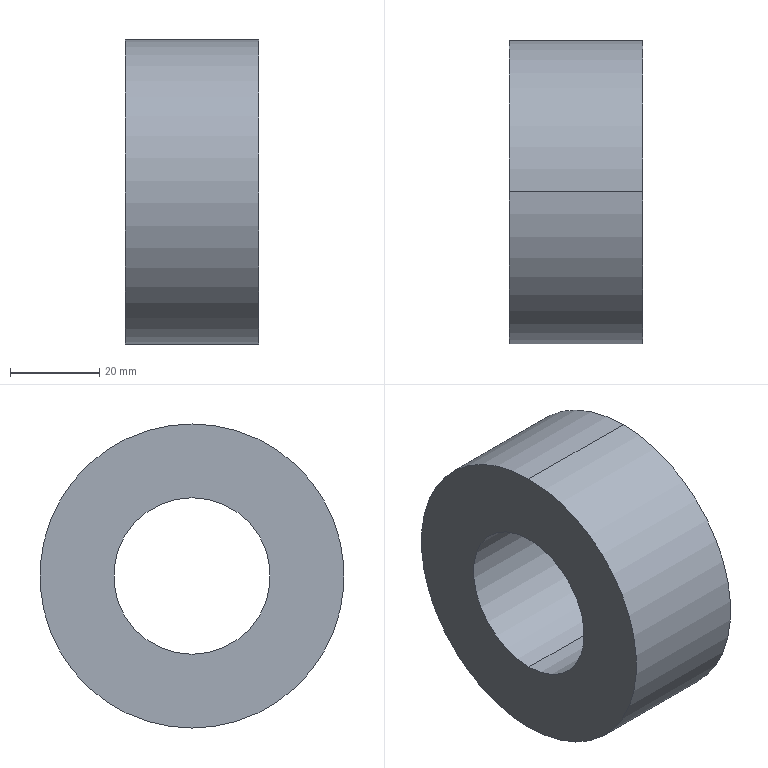Component | SolidWorks | SmallThrustBearing-1 | 1 solid | 8 faces | box 29.79 x 68 x 68 mm | volume 79399 mm3 | cylinder 4 | cone 2 | plane 2 | commonest cylinder face diameters 35 x2 68 x2
build123d program:
from build123d import *

# Parameters (mm, degrees)
SKETCH1_R           = 34
SKETCH1_R_2         = 17.5
BOSS_EXTRUDE1_DEPTH = 29.79
CHAMFER1_SIZE       = 1.5


with BuildPart() as part:
    # Sketch1 → Boss-Extrude1 (new body)
    with BuildSketch(Plane(origin=(0, 0, 0), x_dir=(0, 0, -1), z_dir=(1, 0, 0))):
        Circle(SKETCH1_R)
        Circle(SKETCH1_R_2, mode=Mode.SUBTRACT)
    extrude(amount=BOSS_EXTRUDE1_DEPTH)

    # Chamfer1
    chamfer1_edges = [part.edges().sort_by_distance(p)[0] for p in [
        (29.79, 0, 17.5),
    ]]
    chamfer(chamfer1_edges, length=CHAMFER1_SIZE)


solid = part.part

# Placed as in the assembly
solid = solid.moved(Location((459.733, 15.31, -240), (0, 0, 0)))
STEP:
#1=COLOUR_RGB('',0.7922,0.8196,0.9333);
#2=FILL_AREA_STYLE_COLOUR('',#1);
#3=FILL_AREA_STYLE('',(#2));
#4=SURFACE_STYLE_FILL_AREA(#3);
#5=SURFACE_SIDE_STYLE('',(#4));
#6=SURFACE_STYLE_USAGE(.BOTH.,#5);
#7=PRESENTATION_STYLE_ASSIGNMENT((#6));
#8=CARTESIAN_POINT('',(19.213,0.6028,-8.76));
#9=VERTEX_POINT('',#8);
#10=CARTESIAN_POINT('',(19.213,0.6028,-10.138));
#11=VERTEX_POINT('',#10);
#12=CARTESIAN_POINT('',(19.213,0.6028,-9.449));
#13=DIRECTION('',(1.,0.,0.));
#14=DIRECTION('',(0.,0.,-1.));
#15=AXIS2_PLACEMENT_3D('',#12,#13,#14);
#16=CIRCLE('',#15,0.689);
#17=EDGE_CURVE('',#9,#11,#16,.T.);
#18=ORIENTED_EDGE('',*,*,#17,.F.);
#19=CARTESIAN_POINT('',(19.273,0.6028,-8.701));
#20=VERTEX_POINT('',#19);
#21=CARTESIAN_POINT('',(19.213,0.6028,-8.76));
#22=DIRECTION('',(0.7071,0.,0.7071));
#23=VECTOR('',#22,39.37);
#24=LINE('',#21,#23);
#25=EDGE_CURVE('',#9,#20,#24,.T.);
#26=ORIENTED_EDGE('',*,*,#25,.T.);
#27=CARTESIAN_POINT('',(19.273,0.6028,-10.197));
#28=VERTEX_POINT('',#27);
#29=CARTESIAN_POINT('',(19.273,0.6028,-9.449));
#30=DIRECTION('',(-1.,0.,0.));
#31=DIRECTION('',(0.,0.,-1.));
#32=AXIS2_PLACEMENT_3D('',#29,#30,#31);
#33=CIRCLE('',#32,0.748);
#34=EDGE_CURVE('',#28,#20,#33,.T.);
#35=ORIENTED_EDGE('',*,*,#34,.F.);
#36=CARTESIAN_POINT('',(19.213,0.6028,-10.138));
#37=DIRECTION('',(0.7071,0.,-0.7071));
#38=VECTOR('',#37,39.37);
#39=LINE('',#36,#38);
#40=EDGE_CURVE('',#11,#28,#39,.T.);
#41=ORIENTED_EDGE('',*,*,#40,.F.);
#42=EDGE_LOOP('',(#18,#26,#35,#41));
#43=FACE_OUTER_BOUND('',#42,.T.);
#44=CARTESIAN_POINT('',(19.213,0.6028,-9.449));
#45=DIRECTION('',(1.,0.,0.));
#46=DIRECTION('',(0.,0.,-1.));
#47=AXIS2_PLACEMENT_3D('',#44,#45,#46);
#48=CONICAL_SURFACE('',#47,0.689,0.7854);
#49=ADVANCED_FACE('',(#43),#48,.F.);
#50=ORIENTED_EDGE('',*,*,#17,.T.);
#51=CARTESIAN_POINT('',(18.1,0.6028,-10.138));
#52=VERTEX_POINT('',#51);
#53=CARTESIAN_POINT('',(19.273,0.6028,-10.138));
#54=DIRECTION('',(-1.,0.,0.));
#55=VECTOR('',#54,39.37);
#56=LINE('',#53,#55);
#57=EDGE_CURVE('',#11,#52,#56,.T.);
#58=ORIENTED_EDGE('',*,*,#57,.T.);
#59=CARTESIAN_POINT('',(18.1,0.6028,-8.76));
#60=VERTEX_POINT('',#59);
#61=CARTESIAN_POINT('',(18.1,0.6028,-9.449));
#62=DIRECTION('',(1.,0.,0.));
#63=DIRECTION('',(0.,0.,-1.));
#64=AXIS2_PLACEMENT_3D('',#61,#62,#63);
#65=CIRCLE('',#64,0.689);
#66=EDGE_CURVE('',#60,#52,#65,.T.);
#67=ORIENTED_EDGE('',*,*,#66,.F.);
#68=CARTESIAN_POINT('',(19.273,0.6028,-8.76));
#69=DIRECTION('',(-1.,0.,0.));
#70=VECTOR('',#69,39.37);
#71=LINE('',#68,#70);
#72=EDGE_CURVE('',#9,#60,#71,.T.);
#73=ORIENTED_EDGE('',*,*,#72,.F.);
#74=EDGE_LOOP('',(#50,#58,#67,#73));
#75=FACE_OUTER_BOUND('',#74,.T.);
#76=CARTESIAN_POINT('',(19.273,0.6028,-9.449));
#77=DIRECTION('',(-1.,0.,0.));
#78=DIRECTION('',(0.,0.,1.));
#79=AXIS2_PLACEMENT_3D('',#76,#77,#78);
#80=CYLINDRICAL_SURFACE('',#79,0.689);
#81=ADVANCED_FACE('',(#75),#80,.F.);
#82=CARTESIAN_POINT('',(19.273,0.6028,-10.787));
#83=VERTEX_POINT('',#82);
#84=CARTESIAN_POINT('',(19.273,0.6028,-8.11));
#85=VERTEX_POINT('',#84);
#86=CARTESIAN_POINT('',(19.273,0.6028,-9.449));
#87=DIRECTION('',(1.,0.,0.));
#88=DIRECTION('',(0.,0.,-1.));
#89=AXIS2_PLACEMENT_3D('',#86,#87,#88);
#90=CIRCLE('',#89,1.339);
#91=EDGE_CURVE('',#83,#85,#90,.T.);
#92=ORIENTED_EDGE('',*,*,#91,.F.);
#93=CARTESIAN_POINT('',(18.1,0.6028,-10.787));
#94=VERTEX_POINT('',#93);
#95=CARTESIAN_POINT('',(19.273,0.6028,-10.787));
#96=DIRECTION('',(-1.,0.,0.));
#97=VECTOR('',#96,39.37);
#98=LINE('',#95,#97);
#99=EDGE_CURVE('',#83,#94,#98,.T.);
#100=ORIENTED_EDGE('',*,*,#99,.T.);
#101=CARTESIAN_POINT('',(18.1,0.6028,-8.11));
#102=VERTEX_POINT('',#101);
#103=CARTESIAN_POINT('',(18.1,0.6028,-9.449));
#104=DIRECTION('',(1.,0.,0.));
#105=DIRECTION('',(0.,0.,-1.));
#106=AXIS2_PLACEMENT_3D('',#103,#104,#105);
#107=CIRCLE('',#106,1.339);
#108=EDGE_CURVE('',#94,#102,#107,.T.);
#109=ORIENTED_EDGE('',*,*,#108,.T.);
#110=CARTESIAN_POINT('',(19.273,0.6028,-8.11));
#111=DIRECTION('',(-1.,0.,0.));
#112=VECTOR('',#111,39.37);
#113=LINE('',#110,#112);
#114=EDGE_CURVE('',#85,#102,#113,.T.);
#115=ORIENTED_EDGE('',*,*,#114,.F.);
#116=EDGE_LOOP('',(#92,#100,#109,#115));
#117=FACE_OUTER_BOUND('',#116,.T.);
#118=CARTESIAN_POINT('',(19.273,0.6028,-9.449));
#119=DIRECTION('',(-1.,0.,0.));
#120=DIRECTION('',(0.,0.,1.));
#121=AXIS2_PLACEMENT_3D('',#118,#119,#120);
#122=CYLINDRICAL_SURFACE('',#121,1.339);
#123=ADVANCED_FACE('',(#117),#122,.T.);
#124=ORIENTED_EDGE('',*,*,#34,.T.);
#125=CARTESIAN_POINT('',(19.273,0.6028,-9.449));
#126=DIRECTION('',(-1.,0.,0.));
#127=DIRECTION('',(0.,0.,-1.));
#128=AXIS2_PLACEMENT_3D('',#125,#126,#127);
#129=CIRCLE('',#128,0.748);
#130=EDGE_CURVE('',#20,#28,#129,.T.);
#131=ORIENTED_EDGE('',*,*,#130,.T.);
#132=EDGE_LOOP('',(#124,#131));
#133=FACE_BOUND('',#132,.T.);
#134=CARTESIAN_POINT('',(19.273,0.6028,-9.449));
#135=DIRECTION('',(1.,0.,0.));
#136=DIRECTION('',(0.,0.,-1.));
#137=AXIS2_PLACEMENT_3D('',#134,#135,#136);
#138=CIRCLE('',#137,1.339);
#139=EDGE_CURVE('',#85,#83,#138,.T.);
#140=ORIENTED_EDGE('',*,*,#139,.T.);
#141=ORIENTED_EDGE('',*,*,#91,.T.);
#142=EDGE_LOOP('',(#140,#141));
#143=FACE_OUTER_BOUND('',#142,.T.);
#144=CARTESIAN_POINT('',(19.273,0.6028,-9.449));
#145=DIRECTION('',(1.,0.,0.));
#146=DIRECTION('',(0.,0.,-1.));
#147=AXIS2_PLACEMENT_3D('',#144,#145,#146);
#148=PLANE('',#147);
#149=ADVANCED_FACE('',(#133,#143),#148,.T.);
#150=CARTESIAN_POINT('',(18.1,0.6028,-9.449));
#151=DIRECTION('',(1.,0.,0.));
#152=DIRECTION('',(0.,0.,-1.));
#153=AXIS2_PLACEMENT_3D('',#150,#151,#152);
#154=CIRCLE('',#153,1.339);
#155=EDGE_CURVE('',#102,#94,#154,.T.);
#156=ORIENTED_EDGE('',*,*,#155,.F.);
#157=ORIENTED_EDGE('',*,*,#108,.F.);
#158=EDGE_LOOP('',(#156,#157));
#159=FACE_OUTER_BOUND('',#158,.T.);
#160=ORIENTED_EDGE('',*,*,#66,.T.);
#161=CARTESIAN_POINT('',(18.1,0.6028,-9.449));
#162=DIRECTION('',(1.,0.,0.));
#163=DIRECTION('',(0.,0.,-1.));
#164=AXIS2_PLACEMENT_3D('',#161,#162,#163);
#165=CIRCLE('',#164,0.689);
#166=EDGE_CURVE('',#52,#60,#165,.T.);
#167=ORIENTED_EDGE('',*,*,#166,.T.);
#168=EDGE_LOOP('',(#160,#167));
#169=FACE_BOUND('',#168,.T.);
#170=CARTESIAN_POINT('',(18.1,0.6028,-9.449));
#171=DIRECTION('',(1.,0.,0.));
#172=DIRECTION('',(0.,0.,-1.));
#173=AXIS2_PLACEMENT_3D('',#170,#171,#172);
#174=PLANE('',#173);
#175=ADVANCED_FACE('',(#159,#169),#174,.F.);
#176=ORIENTED_EDGE('',*,*,#99,.F.);
#177=ORIENTED_EDGE('',*,*,#139,.F.);
#178=ORIENTED_EDGE('',*,*,#114,.T.);
#179=ORIENTED_EDGE('',*,*,#155,.T.);
#180=EDGE_LOOP('',(#176,#177,#178,#179));
#181=FACE_OUTER_BOUND('',#180,.T.);
#182=CARTESIAN_POINT('',(19.273,0.6028,-9.449));
#183=DIRECTION('',(-1.,0.,0.));
#184=DIRECTION('',(0.,0.,1.));
#185=AXIS2_PLACEMENT_3D('',#182,#183,#184);
#186=CYLINDRICAL_SURFACE('',#185,1.339);
#187=ADVANCED_FACE('',(#181),#186,.T.);
#188=ORIENTED_EDGE('',*,*,#57,.F.);
#189=CARTESIAN_POINT('',(19.213,0.6028,-9.449));
#190=DIRECTION('',(1.,0.,0.));
#191=DIRECTION('',(0.,0.,-1.));
#192=AXIS2_PLACEMENT_3D('',#189,#190,#191);
#193=CIRCLE('',#192,0.689);
#194=EDGE_CURVE('',#11,#9,#193,.T.);
#195=ORIENTED_EDGE('',*,*,#194,.T.);
#196=ORIENTED_EDGE('',*,*,#72,.T.);
#197=ORIENTED_EDGE('',*,*,#166,.F.);
#198=EDGE_LOOP('',(#188,#195,#196,#197));
#199=FACE_OUTER_BOUND('',#198,.T.);
#200=CARTESIAN_POINT('',(19.273,0.6028,-9.449));
#201=DIRECTION('',(-1.,0.,0.));
#202=DIRECTION('',(0.,0.,1.));
#203=AXIS2_PLACEMENT_3D('',#200,#201,#202);
#204=CYLINDRICAL_SURFACE('',#203,0.689);
#205=ADVANCED_FACE('',(#199),#204,.F.);
#206=ORIENTED_EDGE('',*,*,#25,.F.);
#207=ORIENTED_EDGE('',*,*,#194,.F.);
#208=ORIENTED_EDGE('',*,*,#40,.T.);
#209=ORIENTED_EDGE('',*,*,#130,.F.);
#210=EDGE_LOOP('',(#206,#207,#208,#209));
#211=FACE_OUTER_BOUND('',#210,.T.);
#212=CARTESIAN_POINT('',(19.213,0.6028,-9.449));
#213=DIRECTION('',(1.,0.,0.));
#214=DIRECTION('',(0.,0.,-1.));
#215=AXIS2_PLACEMENT_3D('',#212,#213,#214);
#216=CONICAL_SURFACE('',#215,0.689,0.7854);
#217=ADVANCED_FACE('',(#211),#216,.F.);
#218=CLOSED_SHELL('',(#49,#81,#123,#149,#175,#187,#205,#217));
#219=MANIFOLD_SOLID_BREP('',#218);
#220=STYLED_ITEM('',(#7),#219);
#221=(LENGTH_UNIT()NAMED_UNIT(*)SI_UNIT($,.METRE.));
#222=LENGTH_MEASURE_WITH_UNIT(LENGTH_MEASURE(0.0254),#221);
#223=DIMENSIONAL_EXPONENTS(1.,0.,0.,0.,0.,0.,0.);
#224=(CONVERSION_BASED_UNIT('',#222)LENGTH_UNIT()NAMED_UNIT(#223));
#225=UNCERTAINTY_MEASURE_WITH_UNIT(LENGTH_MEASURE(0.00001),#224,'','');
#226=(NAMED_UNIT(*)PLANE_ANGLE_UNIT()SI_UNIT($,.RADIAN.));
#227=(NAMED_UNIT(*)SI_UNIT($,.STERADIAN.)SOLID_ANGLE_UNIT());
#228=(GEOMETRIC_REPRESENTATION_CONTEXT(3)GLOBAL_UNCERTAINTY_ASSIGNED_CONTEXT((#225))GLOBAL_UNIT_ASSIGNED_CONTEXT((#224,#226,#227))REPRESENTATION_CONTEXT('',''));
#229=MECHANICAL_DESIGN_GEOMETRIC_PRESENTATION_REPRESENTATION('',(#220),#228);
#230=CARTESIAN_POINT('',(0.,0.,0.));
#231=DIRECTION('',(0.,0.,1.));
#232=DIRECTION('',(1.,0.,0.));
#233=AXIS2_PLACEMENT_3D('',#230,#231,#232);
#234=(LENGTH_UNIT()NAMED_UNIT(*)SI_UNIT($,.METRE.));
#235=LENGTH_MEASURE_WITH_UNIT(LENGTH_MEASURE(0.0254),#234);
#236=DIMENSIONAL_EXPONENTS(1.,0.,0.,0.,0.,0.,0.);
#237=(CONVERSION_BASED_UNIT('',#235)LENGTH_UNIT()NAMED_UNIT(#236));
#238=UNCERTAINTY_MEASURE_WITH_UNIT(LENGTH_MEASURE(0.00001),#237,'','');
#239=(NAMED_UNIT(*)PLANE_ANGLE_UNIT()SI_UNIT($,.RADIAN.));
#240=(NAMED_UNIT(*)SI_UNIT($,.STERADIAN.)SOLID_ANGLE_UNIT());
#241=(GEOMETRIC_REPRESENTATION_CONTEXT(3)GLOBAL_UNCERTAINTY_ASSIGNED_CONTEXT((#238))GLOBAL_UNIT_ASSIGNED_CONTEXT((#237,#239,#240))REPRESENTATION_CONTEXT('',''));
#242=ADVANCED_BREP_SHAPE_REPRESENTATION('',(#219,#233),#241);
#243=PRESENTATION_LAYER_ASSIGNMENT('','',(#220));